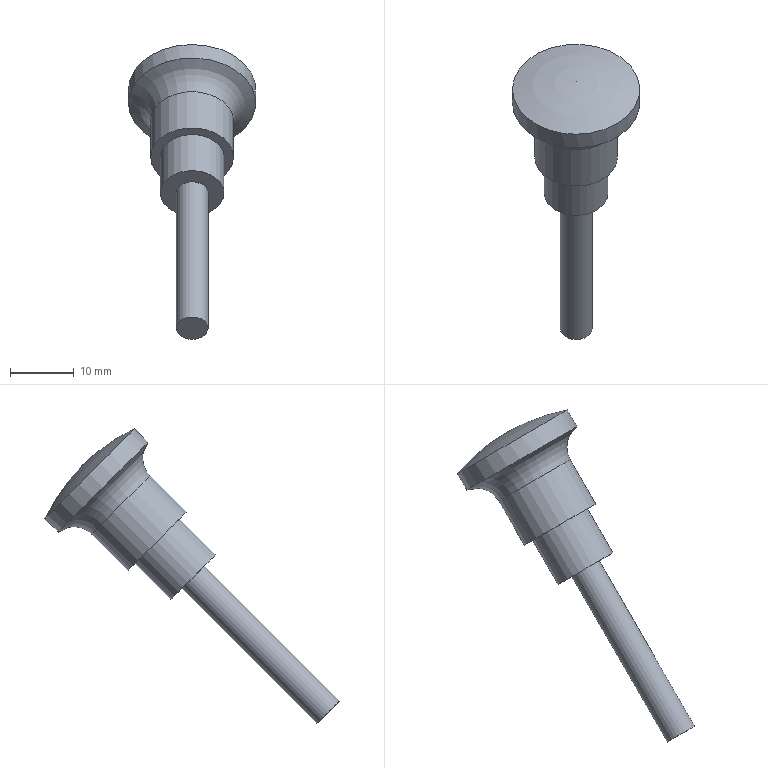Component | NX | YOUBIAO | 1 solid | 9 faces | box 20 x 46.32 x 46.32 mm | volume 4178 mm3 | cylinder 4 | plane 3 | sphere 1 | torus 1 | commonest cylinder face diameters 5 x1 10 x1 20 x1 13 x1
STEP:
#1=CARTESIAN_POINT('',(0.,0.,0.));
#2=DIRECTION('',(0.,0.,1.));
#3=DIRECTION('',(1.,0.,0.));
#4=AXIS2_PLACEMENT_3D('',#1,#2,#3);
#5=CARTESIAN_POINT('',(2.5,317.929,-155.071));
#6=VERTEX_POINT('',#5);
#7=CARTESIAN_POINT('',(0.,317.929,-155.071));
#8=DIRECTION('',(0.,0.7071,0.7071));
#9=DIRECTION('',(1.,0.,0.));
#10=AXIS2_PLACEMENT_3D('',#7,#8,#9);
#11=CIRCLE('',#10,2.5);
#12=CARTESIAN_POINT('',(0.,317.929,-155.071));
#13=DIRECTION('',(0.,-0.7071,-0.7071));
#14=DIRECTION('',(-1.,0.,0.));
#15=AXIS2_PLACEMENT_3D('',#12,#13,#14);
#16=CYLINDRICAL_SURFACE('',#15,2.5);
#17=CARTESIAN_POINT('',(9.425,0.));
#18=DIRECTION('',(-1.,0.));
#19=VECTOR('',#18,1.);
#20=LINE('',#17,#19);
#21=(GEOMETRIC_REPRESENTATION_CONTEXT(2)PARAMETRIC_REPRESENTATION_CONTEXT()REPRESENTATION_CONTEXT('',''));
#22=DEFINITIONAL_REPRESENTATION('',(#20),#21);
#23=PCURVE('',#16,#22);
#24=CARTESIAN_POINT('',(0.,317.929,-155.071));
#25=DIRECTION('',(0.,0.7071,0.7071));
#26=DIRECTION('',(1.,0.,0.));
#27=AXIS2_PLACEMENT_3D('',#24,#25,#26);
#28=PLANE('',#27);
#29=CARTESIAN_POINT('',(0.,0.));
#30=DIRECTION('',(1.,0.));
#31=AXIS2_PLACEMENT_2D('',#29,#30);
#32=CIRCLE('',#31,2.5);
#33=(GEOMETRIC_REPRESENTATION_CONTEXT(2)PARAMETRIC_REPRESENTATION_CONTEXT()REPRESENTATION_CONTEXT('',''));
#34=DEFINITIONAL_REPRESENTATION('',(#32),#33);
#35=PCURVE('',#28,#34);
#36=SURFACE_CURVE('',#11,(#23,#35),.PCURVE_S1.);
#37=EDGE_CURVE('',#6,#6,#36,.T.);
#38=ORIENTED_EDGE('',*,*,#37,.F.);
#39=CARTESIAN_POINT('',(2.5,296.716,-176.284));
#40=VERTEX_POINT('',#39);
#41=CARTESIAN_POINT('',(2.5,317.929,-155.071));
#42=CARTESIAN_POINT('',(2.5,296.716,-176.284));
#43=B_SPLINE_CURVE_WITH_KNOTS('',1,(#41,#42),.UNSPECIFIED.,.F.,.F.,(2,2),(0.,30.),.PIECEWISE_BEZIER_KNOTS.);
#44=CARTESIAN_POINT('',(9.425,0.));
#45=DIRECTION('',(0.,1.));
#46=VECTOR('',#45,1.);
#47=LINE('',#44,#46);
#48=(GEOMETRIC_REPRESENTATION_CONTEXT(2)PARAMETRIC_REPRESENTATION_CONTEXT()REPRESENTATION_CONTEXT('',''));
#49=DEFINITIONAL_REPRESENTATION('',(#47),#48);
#50=PCURVE('',#16,#49);
#51=CARTESIAN_POINT('',(3.142,0.));
#52=DIRECTION('',(0.,1.));
#53=VECTOR('',#52,1.);
#54=LINE('',#51,#53);
#55=(GEOMETRIC_REPRESENTATION_CONTEXT(2)PARAMETRIC_REPRESENTATION_CONTEXT()REPRESENTATION_CONTEXT('',''));
#56=DEFINITIONAL_REPRESENTATION('',(#54),#55);
#57=PCURVE('',#16,#56);
#58=SEAM_CURVE('',#43,(#50,#57),.PCURVE_S1.);
#59=EDGE_CURVE('',#6,#40,#58,.T.);
#60=ORIENTED_EDGE('',*,*,#59,.T.);
#61=CARTESIAN_POINT('',(0.,296.716,-176.284));
#62=DIRECTION('',(0.,0.7071,0.7071));
#63=DIRECTION('',(1.,0.,0.));
#64=AXIS2_PLACEMENT_3D('',#61,#62,#63);
#65=CIRCLE('',#64,2.5);
#66=CARTESIAN_POINT('',(9.425,30.));
#67=DIRECTION('',(-1.,0.));
#68=VECTOR('',#67,1.);
#69=LINE('',#66,#68);
#70=(GEOMETRIC_REPRESENTATION_CONTEXT(2)PARAMETRIC_REPRESENTATION_CONTEXT()REPRESENTATION_CONTEXT('',''));
#71=DEFINITIONAL_REPRESENTATION('',(#69),#70);
#72=PCURVE('',#16,#71);
#73=CARTESIAN_POINT('',(0.,296.716,-176.284));
#74=DIRECTION('',(0.,0.7071,0.7071));
#75=DIRECTION('',(1.,0.,0.));
#76=AXIS2_PLACEMENT_3D('',#73,#74,#75);
#77=PLANE('',#76);
#78=CARTESIAN_POINT('',(0.,0.));
#79=DIRECTION('',(1.,0.));
#80=AXIS2_PLACEMENT_2D('',#78,#79);
#81=CIRCLE('',#80,2.5);
#82=(GEOMETRIC_REPRESENTATION_CONTEXT(2)PARAMETRIC_REPRESENTATION_CONTEXT()REPRESENTATION_CONTEXT('',''));
#83=DEFINITIONAL_REPRESENTATION('',(#81),#82);
#84=PCURVE('',#77,#83);
#85=SURFACE_CURVE('',#65,(#72,#84),.PCURVE_S1.);
#86=EDGE_CURVE('',#40,#40,#85,.T.);
#87=ORIENTED_EDGE('',*,*,#86,.T.);
#88=ORIENTED_EDGE('',*,*,#59,.F.);
#89=EDGE_LOOP('',(#38,#60,#87,#88));
#90=FACE_BOUND('',#89,.T.);
#91=ADVANCED_FACE('',(#90),#16,.T.);
#92=ORIENTED_EDGE('',*,*,#86,.F.);
#93=EDGE_LOOP('',(#92));
#94=FACE_BOUND('',#93,.T.);
#95=ADVANCED_FACE('',(#94),#77,.F.);
#96=CARTESIAN_POINT('',(5.,317.929,-155.071));
#97=VERTEX_POINT('',#96);
#98=CARTESIAN_POINT('',(0.,317.929,-155.071));
#99=DIRECTION('',(0.,0.7071,0.7071));
#100=DIRECTION('',(1.,0.,0.));
#101=AXIS2_PLACEMENT_3D('',#98,#99,#100);
#102=CIRCLE('',#101,5.);
#103=CARTESIAN_POINT('',(0.,0.));
#104=DIRECTION('',(1.,0.));
#105=AXIS2_PLACEMENT_2D('',#103,#104);
#106=CIRCLE('',#105,5.);
#107=(GEOMETRIC_REPRESENTATION_CONTEXT(2)PARAMETRIC_REPRESENTATION_CONTEXT()REPRESENTATION_CONTEXT('',''));
#108=DEFINITIONAL_REPRESENTATION('',(#106),#107);
#109=PCURVE('',#28,#108);
#110=CARTESIAN_POINT('',(0.,323.586,-149.414));
#111=DIRECTION('',(0.,-0.7071,-0.7071));
#112=DIRECTION('',(-1.,0.,0.));
#113=AXIS2_PLACEMENT_3D('',#110,#111,#112);
#114=CYLINDRICAL_SURFACE('',#113,5.);
#115=CARTESIAN_POINT('',(9.425,8.));
#116=DIRECTION('',(-1.,0.));
#117=VECTOR('',#116,1.);
#118=LINE('',#115,#117);
#119=(GEOMETRIC_REPRESENTATION_CONTEXT(2)PARAMETRIC_REPRESENTATION_CONTEXT()REPRESENTATION_CONTEXT('',''));
#120=DEFINITIONAL_REPRESENTATION('',(#118),#119);
#121=PCURVE('',#114,#120);
#122=SURFACE_CURVE('',#102,(#109,#121),.PCURVE_S1.);
#123=EDGE_CURVE('',#97,#97,#122,.T.);
#124=ORIENTED_EDGE('',*,*,#123,.F.);
#125=EDGE_LOOP('',(#124));
#126=FACE_BOUND('',#125,.T.);
#127=ORIENTED_EDGE('',*,*,#37,.T.);
#128=EDGE_LOOP('',(#127));
#129=FACE_BOUND('',#128,.T.);
#130=ADVANCED_FACE('',(#126,#129),#28,.F.);
#131=CARTESIAN_POINT('',(5.,323.586,-149.414));
#132=VERTEX_POINT('',#131);
#133=CARTESIAN_POINT('',(0.,323.586,-149.414));
#134=DIRECTION('',(0.,0.7071,0.7071));
#135=DIRECTION('',(1.,0.,0.));
#136=AXIS2_PLACEMENT_3D('',#133,#134,#135);
#137=CIRCLE('',#136,5.);
#138=CARTESIAN_POINT('',(9.425,0.));
#139=DIRECTION('',(-1.,0.));
#140=VECTOR('',#139,1.);
#141=LINE('',#138,#140);
#142=(GEOMETRIC_REPRESENTATION_CONTEXT(2)PARAMETRIC_REPRESENTATION_CONTEXT()REPRESENTATION_CONTEXT('',''));
#143=DEFINITIONAL_REPRESENTATION('',(#141),#142);
#144=PCURVE('',#114,#143);
#145=CARTESIAN_POINT('',(0.,323.586,-149.414));
#146=DIRECTION('',(0.,-0.7071,-0.7071));
#147=DIRECTION('',(-1.,0.,0.));
#148=AXIS2_PLACEMENT_3D('',#145,#146,#147);
#149=PLANE('',#148);
#150=CARTESIAN_POINT('',(-5.,0.));
#151=CARTESIAN_POINT('',(-5.,8.66));
#152=CARTESIAN_POINT('',(2.5,4.33));
#153=CARTESIAN_POINT('',(10.,0.));
#154=CARTESIAN_POINT('',(2.5,-4.33));
#155=CARTESIAN_POINT('',(-5.,-8.66));
#156=CARTESIAN_POINT('',(-5.,0.));
#157=(BOUNDED_CURVE()B_SPLINE_CURVE(2,(#150,#151,#152,#153,#154,#155,#156),.UNSPECIFIED.,.T.,.F.)B_SPLINE_CURVE_WITH_KNOTS((1,2,2,2,2,1),(-2.094,0.,2.094,4.189,6.283,8.378),.UNSPECIFIED.)CURVE()GEOMETRIC_REPRESENTATION_ITEM()RATIONAL_B_SPLINE_CURVE((1.,0.5,1.,0.5,1.,0.5,1.))REPRESENTATION_ITEM(''));
#158=(GEOMETRIC_REPRESENTATION_CONTEXT(2)PARAMETRIC_REPRESENTATION_CONTEXT()REPRESENTATION_CONTEXT('',''));
#159=DEFINITIONAL_REPRESENTATION('',(#157),#158);
#160=PCURVE('',#149,#159);
#161=SURFACE_CURVE('',#137,(#144,#160),.PCURVE_S1.);
#162=EDGE_CURVE('',#132,#132,#161,.T.);
#163=ORIENTED_EDGE('',*,*,#162,.F.);
#164=CARTESIAN_POINT('',(5.,323.586,-149.414));
#165=CARTESIAN_POINT('',(5.,317.929,-155.071));
#166=B_SPLINE_CURVE_WITH_KNOTS('',1,(#164,#165),.UNSPECIFIED.,.F.,.F.,(2,2),(0.,8.),.PIECEWISE_BEZIER_KNOTS.);
#167=CARTESIAN_POINT('',(9.425,0.));
#168=DIRECTION('',(0.,1.));
#169=VECTOR('',#168,1.);
#170=LINE('',#167,#169);
#171=(GEOMETRIC_REPRESENTATION_CONTEXT(2)PARAMETRIC_REPRESENTATION_CONTEXT()REPRESENTATION_CONTEXT('',''));
#172=DEFINITIONAL_REPRESENTATION('',(#170),#171);
#173=PCURVE('',#114,#172);
#174=CARTESIAN_POINT('',(3.142,0.));
#175=DIRECTION('',(0.,1.));
#176=VECTOR('',#175,1.);
#177=LINE('',#174,#176);
#178=(GEOMETRIC_REPRESENTATION_CONTEXT(2)PARAMETRIC_REPRESENTATION_CONTEXT()REPRESENTATION_CONTEXT('',''));
#179=DEFINITIONAL_REPRESENTATION('',(#177),#178);
#180=PCURVE('',#114,#179);
#181=SEAM_CURVE('',#166,(#173,#180),.PCURVE_S1.);
#182=EDGE_CURVE('',#132,#97,#181,.T.);
#183=ORIENTED_EDGE('',*,*,#182,.T.);
#184=ORIENTED_EDGE('',*,*,#123,.T.);
#185=ORIENTED_EDGE('',*,*,#182,.F.);
#186=EDGE_LOOP('',(#163,#183,#184,#185));
#187=FACE_BOUND('',#186,.T.);
#188=ADVANCED_FACE('',(#187),#114,.T.);
#189=ORIENTED_EDGE('',*,*,#162,.T.);
#190=EDGE_LOOP('',(#189));
#191=FACE_BOUND('',#190,.T.);
#192=CARTESIAN_POINT('',(-6.5,323.586,-149.414));
#193=VERTEX_POINT('',#192);
#194=CARTESIAN_POINT('',(0.,323.586,-149.414));
#195=DIRECTION('',(0.,-0.7071,-0.7071));
#196=DIRECTION('',(-1.,0.,0.));
#197=AXIS2_PLACEMENT_3D('',#194,#195,#196);
#198=CIRCLE('',#197,6.5);
#199=CARTESIAN_POINT('',(0.,0.));
#200=DIRECTION('',(1.,0.));
#201=AXIS2_PLACEMENT_2D('',#199,#200);
#202=CIRCLE('',#201,6.5);
#203=(GEOMETRIC_REPRESENTATION_CONTEXT(2)PARAMETRIC_REPRESENTATION_CONTEXT()REPRESENTATION_CONTEXT('',''));
#204=DEFINITIONAL_REPRESENTATION('',(#202),#203);
#205=PCURVE('',#149,#204);
#206=CARTESIAN_POINT('',(0.,323.586,-149.414));
#207=DIRECTION('',(0.,-0.7071,-0.7071));
#208=DIRECTION('',(-1.,0.,0.));
#209=AXIS2_PLACEMENT_3D('',#206,#207,#208);
#210=CYLINDRICAL_SURFACE('',#209,6.5);
#211=CARTESIAN_POINT('',(0.,0.));
#212=DIRECTION('',(1.,0.));
#213=VECTOR('',#212,1.);
#214=LINE('',#211,#213);
#215=(GEOMETRIC_REPRESENTATION_CONTEXT(2)PARAMETRIC_REPRESENTATION_CONTEXT()REPRESENTATION_CONTEXT('',''));
#216=DEFINITIONAL_REPRESENTATION('',(#214),#215);
#217=PCURVE('',#210,#216);
#218=SURFACE_CURVE('',#198,(#205,#217),.PCURVE_S1.);
#219=EDGE_CURVE('',#193,#193,#218,.T.);
#220=ORIENTED_EDGE('',*,*,#219,.T.);
#221=EDGE_LOOP('',(#220));
#222=FACE_BOUND('',#221,.T.);
#223=ADVANCED_FACE('',(#191,#222),#149,.T.);
#224=CARTESIAN_POINT('',(0.,327.121,-131.737));
#225=VERTEX_POINT('',#224);
#226=CARTESIAN_POINT('',(-10.,334.192,-138.808));
#227=VERTEX_POINT('',#226);
#228=CARTESIAN_POINT('',(0.,334.192,-138.808));
#229=DIRECTION('',(0.,-0.7071,-0.7071));
#230=DIRECTION('',(-1.,0.,0.));
#231=AXIS2_PLACEMENT_3D('',#228,#229,#230);
#232=CIRCLE('',#231,10.);
#233=CARTESIAN_POINT('',(0.,314.192,-158.808));
#234=DIRECTION('',(0.,-0.7071,-0.7071));
#235=DIRECTION('',(0.,-0.7071,0.7071));
#236=AXIS2_PLACEMENT_3D('',#233,#234,#235);
#237=SPHERICAL_SURFACE('',#236,30.);
#238=CARTESIAN_POINT('',(-4.712,-1.231));
#239=CARTESIAN_POINT('',(-4.617,-1.231));
#240=CARTESIAN_POINT('',(-4.427,-1.231));
#241=CARTESIAN_POINT('',(-4.141,-1.231));
#242=CARTESIAN_POINT('',(-3.856,-1.231));
#243=CARTESIAN_POINT('',(-3.57,-1.231));
#244=CARTESIAN_POINT('',(-3.284,-1.231));
#245=CARTESIAN_POINT('',(-2.999,-1.231));
#246=CARTESIAN_POINT('',(-2.713,-1.231));
#247=CARTESIAN_POINT('',(-2.428,-1.231));
#248=CARTESIAN_POINT('',(-2.142,-1.231));
#249=CARTESIAN_POINT('',(-1.856,-1.231));
#250=CARTESIAN_POINT('',(-1.571,-1.231));
#251=CARTESIAN_POINT('',(-1.285,-1.231));
#252=CARTESIAN_POINT('',(-0.9996,-1.231));
#253=CARTESIAN_POINT('',(-0.714,-1.231));
#254=CARTESIAN_POINT('',(-0.4284,-1.231));
#255=CARTESIAN_POINT('',(-0.1428,-1.231));
#256=CARTESIAN_POINT('',(0.1428,-1.231));
#257=CARTESIAN_POINT('',(0.4284,-1.231));
#258=CARTESIAN_POINT('',(0.714,-1.231));
#259=CARTESIAN_POINT('',(0.9996,-1.231));
#260=CARTESIAN_POINT('',(1.285,-1.231));
#261=CARTESIAN_POINT('',(1.476,-1.231));
#262=CARTESIAN_POINT('',(1.571,-1.231));
#263=B_SPLINE_CURVE_WITH_KNOTS('',3,(#238,#239,#240,#241,#242,#243,#244,#245,#246,#247,#248,#249,#250,#251,#252,#253,#254,#255,#256,#257,#258,#259,#260,#261,#262),.UNSPECIFIED.,.F.,.F.,(4,1,1,1,1,1,1,1,1,1,1,1,1,1,1,1,1,1,1,1,1,1,4),(0.,0.2856,0.5712,0.8568,1.142,1.428,1.714,1.999,2.285,2.57,2.856,3.142,3.427,3.713,3.998,4.284,4.57,4.855,5.141,5.426,5.712,5.998,6.283),.QUASI_UNIFORM_KNOTS.);
#264=(GEOMETRIC_REPRESENTATION_CONTEXT(2)PARAMETRIC_REPRESENTATION_CONTEXT()REPRESENTATION_CONTEXT('',''));
#265=DEFINITIONAL_REPRESENTATION('',(#263),#264);
#266=PCURVE('',#237,#265);
#267=CARTESIAN_POINT('',(0.,323.586,-149.414));
#268=DIRECTION('',(0.,-0.7071,-0.7071));
#269=DIRECTION('',(-1.,0.,0.));
#270=AXIS2_PLACEMENT_3D('',#267,#268,#269);
#271=CYLINDRICAL_SURFACE('',#270,10.);
#272=CARTESIAN_POINT('',(0.,-15.));
#273=DIRECTION('',(1.,0.));
#274=VECTOR('',#273,1.);
#275=LINE('',#272,#274);
#276=(GEOMETRIC_REPRESENTATION_CONTEXT(2)PARAMETRIC_REPRESENTATION_CONTEXT()REPRESENTATION_CONTEXT('',''));
#277=DEFINITIONAL_REPRESENTATION('',(#275),#276);
#278=PCURVE('',#271,#277);
#279=SURFACE_CURVE('',#232,(#266,#278),.PCURVE_S1.);
#280=EDGE_CURVE('',#225,#227,#279,.T.);
#281=ORIENTED_EDGE('',*,*,#280,.F.);
#282=CARTESIAN_POINT('',(0.,335.406,-137.594));
#283=VERTEX_POINT('',#282);
#284=CARTESIAN_POINT('',(0.,335.406,-137.594));
#285=CARTESIAN_POINT('',(0.,333.964,-136.153));
#286=CARTESIAN_POINT('',(0.,332.399,-134.833));
#287=CARTESIAN_POINT('',(0.,330.727,-133.65));
#288=CARTESIAN_POINT('',(0.,328.961,-132.615));
#289=CARTESIAN_POINT('',(0.,327.121,-131.737));
#290=B_SPLINE_CURVE_WITH_KNOTS('',5,(#284,#285,#286,#287,#288,#289),.UNSPECIFIED.,.F.,.F.,(6,6),(-1.571,-1.231),.PIECEWISE_BEZIER_KNOTS.);
#291=CARTESIAN_POINT('',(0.,0.));
#292=DIRECTION('',(0.,1.));
#293=VECTOR('',#292,1.);
#294=LINE('',#291,#293);
#295=(GEOMETRIC_REPRESENTATION_CONTEXT(2)PARAMETRIC_REPRESENTATION_CONTEXT()REPRESENTATION_CONTEXT('',''));
#296=DEFINITIONAL_REPRESENTATION('',(#294),#295);
#297=PCURVE('',#237,#296);
#298=CARTESIAN_POINT('',(6.283,0.));
#299=DIRECTION('',(0.,1.));
#300=VECTOR('',#299,1.);
#301=LINE('',#298,#300);
#302=(GEOMETRIC_REPRESENTATION_CONTEXT(2)PARAMETRIC_REPRESENTATION_CONTEXT()REPRESENTATION_CONTEXT('',''));
#303=DEFINITIONAL_REPRESENTATION('',(#301),#302);
#304=PCURVE('',#237,#303);
#305=SEAM_CURVE('',#290,(#297,#304),.PCURVE_S1.);
#306=EDGE_CURVE('',#283,#225,#305,.T.);
#307=ORIENTED_EDGE('',*,*,#306,.F.);
#308=ORIENTED_EDGE('',*,*,#306,.T.);
#309=CARTESIAN_POINT('',(0.,334.192,-138.808));
#310=DIRECTION('',(0.,-0.7071,-0.7071));
#311=DIRECTION('',(-1.,0.,0.));
#312=AXIS2_PLACEMENT_3D('',#309,#310,#311);
#313=CIRCLE('',#312,10.);
#314=CARTESIAN_POINT('',(1.571,-1.231));
#315=CARTESIAN_POINT('',(1.666,-1.231));
#316=CARTESIAN_POINT('',(1.856,-1.231));
#317=CARTESIAN_POINT('',(2.142,-1.231));
#318=CARTESIAN_POINT('',(2.428,-1.231));
#319=CARTESIAN_POINT('',(2.713,-1.231));
#320=CARTESIAN_POINT('',(2.999,-1.231));
#321=CARTESIAN_POINT('',(3.284,-1.231));
#322=CARTESIAN_POINT('',(3.57,-1.231));
#323=CARTESIAN_POINT('',(3.856,-1.231));
#324=CARTESIAN_POINT('',(4.141,-1.231));
#325=CARTESIAN_POINT('',(4.427,-1.231));
#326=CARTESIAN_POINT('',(4.712,-1.231));
#327=CARTESIAN_POINT('',(4.998,-1.231));
#328=CARTESIAN_POINT('',(5.284,-1.231));
#329=CARTESIAN_POINT('',(5.569,-1.231));
#330=CARTESIAN_POINT('',(5.855,-1.231));
#331=CARTESIAN_POINT('',(6.14,-1.231));
#332=CARTESIAN_POINT('',(6.426,-1.231));
#333=CARTESIAN_POINT('',(6.712,-1.231));
#334=CARTESIAN_POINT('',(6.997,-1.231));
#335=CARTESIAN_POINT('',(7.283,-1.231));
#336=CARTESIAN_POINT('',(7.568,-1.231));
#337=CARTESIAN_POINT('',(7.759,-1.231));
#338=CARTESIAN_POINT('',(7.854,-1.231));
#339=B_SPLINE_CURVE_WITH_KNOTS('',3,(#314,#315,#316,#317,#318,#319,#320,#321,#322,#323,#324,#325,#326,#327,#328,#329,#330,#331,#332,#333,#334,#335,#336,#337,#338),.UNSPECIFIED.,.F.,.F.,(4,1,1,1,1,1,1,1,1,1,1,1,1,1,1,1,1,1,1,1,1,1,4),(0.,0.2856,0.5712,0.8568,1.142,1.428,1.714,1.999,2.285,2.57,2.856,3.142,3.427,3.713,3.998,4.284,4.57,4.855,5.141,5.426,5.712,5.998,6.283),.QUASI_UNIFORM_KNOTS.);
#340=(GEOMETRIC_REPRESENTATION_CONTEXT(2)PARAMETRIC_REPRESENTATION_CONTEXT()REPRESENTATION_CONTEXT('',''));
#341=DEFINITIONAL_REPRESENTATION('',(#339),#340);
#342=PCURVE('',#237,#341);
#343=CARTESIAN_POINT('',(0.,-15.));
#344=DIRECTION('',(1.,0.));
#345=VECTOR('',#344,1.);
#346=LINE('',#343,#345);
#347=(GEOMETRIC_REPRESENTATION_CONTEXT(2)PARAMETRIC_REPRESENTATION_CONTEXT()REPRESENTATION_CONTEXT('',''));
#348=DEFINITIONAL_REPRESENTATION('',(#346),#347);
#349=PCURVE('',#271,#348);
#350=SURFACE_CURVE('',#313,(#342,#349),.PCURVE_S1.);
#351=EDGE_CURVE('',#227,#225,#350,.T.);
#352=ORIENTED_EDGE('',*,*,#351,.F.);
#353=EDGE_LOOP('',(#281,#307,#308,#352));
#354=FACE_BOUND('',#353,.T.);
#355=ADVANCED_FACE('',(#354),#237,.T.);
#356=ORIENTED_EDGE('',*,*,#351,.T.);
#357=ORIENTED_EDGE('',*,*,#280,.T.);
#358=CARTESIAN_POINT('',(-10.,332.071,-140.929));
#359=VERTEX_POINT('',#358);
#360=CARTESIAN_POINT('',(-10.,334.192,-138.808));
#361=CARTESIAN_POINT('',(-10.,332.071,-140.929));
#362=B_SPLINE_CURVE_WITH_KNOTS('',1,(#360,#361),.UNSPECIFIED.,.F.,.F.,(2,2),(-15.,-12.),.PIECEWISE_BEZIER_KNOTS.);
#363=CARTESIAN_POINT('',(6.283,0.));
#364=DIRECTION('',(0.,1.));
#365=VECTOR('',#364,1.);
#366=LINE('',#363,#365);
#367=(GEOMETRIC_REPRESENTATION_CONTEXT(2)PARAMETRIC_REPRESENTATION_CONTEXT()REPRESENTATION_CONTEXT('',''));
#368=DEFINITIONAL_REPRESENTATION('',(#366),#367);
#369=PCURVE('',#271,#368);
#370=CARTESIAN_POINT('',(0.,0.));
#371=DIRECTION('',(0.,1.));
#372=VECTOR('',#371,1.);
#373=LINE('',#370,#372);
#374=(GEOMETRIC_REPRESENTATION_CONTEXT(2)PARAMETRIC_REPRESENTATION_CONTEXT()REPRESENTATION_CONTEXT('',''));
#375=DEFINITIONAL_REPRESENTATION('',(#373),#374);
#376=PCURVE('',#271,#375);
#377=SEAM_CURVE('',#362,(#369,#376),.PCURVE_S1.);
#378=EDGE_CURVE('',#227,#359,#377,.T.);
#379=ORIENTED_EDGE('',*,*,#378,.T.);
#380=CARTESIAN_POINT('',(0.,332.071,-140.929));
#381=DIRECTION('',(0.,-0.7071,-0.7071));
#382=DIRECTION('',(-1.,0.,0.));
#383=AXIS2_PLACEMENT_3D('',#380,#381,#382);
#384=CIRCLE('',#383,10.);
#385=CARTESIAN_POINT('',(0.,-12.));
#386=DIRECTION('',(1.,0.));
#387=VECTOR('',#386,1.);
#388=LINE('',#385,#387);
#389=(GEOMETRIC_REPRESENTATION_CONTEXT(2)PARAMETRIC_REPRESENTATION_CONTEXT()REPRESENTATION_CONTEXT('',''));
#390=DEFINITIONAL_REPRESENTATION('',(#388),#389);
#391=PCURVE('',#271,#390);
#392=CARTESIAN_POINT('',(0.,329.265,-143.735));
#393=DIRECTION('',(0.,-0.7071,-0.7071));
#394=DIRECTION('',(-1.,0.,0.));
#395=AXIS2_PLACEMENT_3D('',#392,#393,#394);
#396=TOROIDAL_SURFACE('',#395,10.5,4.);
#397=CARTESIAN_POINT('',(0.,4.587));
#398=DIRECTION('',(1.,0.));
#399=VECTOR('',#398,1.);
#400=LINE('',#397,#399);
#401=(GEOMETRIC_REPRESENTATION_CONTEXT(2)PARAMETRIC_REPRESENTATION_CONTEXT()REPRESENTATION_CONTEXT('',''));
#402=DEFINITIONAL_REPRESENTATION('',(#400),#401);
#403=PCURVE('',#396,#402);
#404=SURFACE_CURVE('',#384,(#391,#403),.PCURVE_S1.);
#405=EDGE_CURVE('',#359,#359,#404,.T.);
#406=ORIENTED_EDGE('',*,*,#405,.F.);
#407=ORIENTED_EDGE('',*,*,#378,.F.);
#408=EDGE_LOOP('',(#356,#357,#379,#406,#407));
#409=FACE_BOUND('',#408,.T.);
#410=ADVANCED_FACE('',(#409),#271,.T.);
#411=ORIENTED_EDGE('',*,*,#405,.F.);
#412=CARTESIAN_POINT('',(-6.5,329.265,-143.735));
#413=VERTEX_POINT('',#412);
#414=CARTESIAN_POINT('',(-6.5,329.265,-143.735));
#415=CARTESIAN_POINT('',(-6.5,329.958,-143.042));
#416=CARTESIAN_POINT('',(-6.786,330.637,-142.363));
#417=CARTESIAN_POINT('',(-7.34,331.236,-141.764));
#418=CARTESIAN_POINT('',(-8.111,331.699,-141.301));
#419=CARTESIAN_POINT('',(-9.027,331.984,-141.016));
#420=CARTESIAN_POINT('',(-10.,332.071,-140.929));
#421=(BOUNDED_CURVE()B_SPLINE_CURVE(6,(#414,#415,#416,#417,#418,#419,#420),.UNSPECIFIED.,.F.,.F.)B_SPLINE_CURVE_WITH_KNOTS((7,7),(3.142,4.587),.PIECEWISE_BEZIER_KNOTS.)CURVE()GEOMETRIC_REPRESENTATION_ITEM()RATIONAL_B_SPLINE_CURVE((1.027,1.009,0.9982,0.9949,0.9982,1.009,1.027))REPRESENTATION_ITEM(''));
#422=CARTESIAN_POINT('',(0.,0.));
#423=DIRECTION('',(0.,1.));
#424=VECTOR('',#423,1.);
#425=LINE('',#422,#424);
#426=(GEOMETRIC_REPRESENTATION_CONTEXT(2)PARAMETRIC_REPRESENTATION_CONTEXT()REPRESENTATION_CONTEXT('',''));
#427=DEFINITIONAL_REPRESENTATION('',(#425),#426);
#428=PCURVE('',#396,#427);
#429=CARTESIAN_POINT('',(6.283,0.));
#430=DIRECTION('',(0.,1.));
#431=VECTOR('',#430,1.);
#432=LINE('',#429,#431);
#433=(GEOMETRIC_REPRESENTATION_CONTEXT(2)PARAMETRIC_REPRESENTATION_CONTEXT()REPRESENTATION_CONTEXT('',''));
#434=DEFINITIONAL_REPRESENTATION('',(#432),#433);
#435=PCURVE('',#396,#434);
#436=SEAM_CURVE('',#421,(#428,#435),.PCURVE_S1.);
#437=EDGE_CURVE('',#413,#359,#436,.T.);
#438=ORIENTED_EDGE('',*,*,#437,.F.);
#439=CARTESIAN_POINT('',(0.,329.265,-143.735));
#440=DIRECTION('',(0.,-0.7071,-0.7071));
#441=DIRECTION('',(-1.,0.,0.));
#442=AXIS2_PLACEMENT_3D('',#439,#440,#441);
#443=CIRCLE('',#442,6.5);
#444=CARTESIAN_POINT('',(0.,3.142));
#445=DIRECTION('',(1.,0.));
#446=VECTOR('',#445,1.);
#447=LINE('',#444,#446);
#448=(GEOMETRIC_REPRESENTATION_CONTEXT(2)PARAMETRIC_REPRESENTATION_CONTEXT()REPRESENTATION_CONTEXT('',''));
#449=DEFINITIONAL_REPRESENTATION('',(#447),#448);
#450=PCURVE('',#396,#449);
#451=CARTESIAN_POINT('',(0.,-8.031));
#452=DIRECTION('',(1.,0.));
#453=VECTOR('',#452,1.);
#454=LINE('',#451,#453);
#455=(GEOMETRIC_REPRESENTATION_CONTEXT(2)PARAMETRIC_REPRESENTATION_CONTEXT()REPRESENTATION_CONTEXT('',''));
#456=DEFINITIONAL_REPRESENTATION('',(#454),#455);
#457=PCURVE('',#210,#456);
#458=SURFACE_CURVE('',#443,(#450,#457),.PCURVE_S1.);
#459=EDGE_CURVE('',#413,#413,#458,.T.);
#460=ORIENTED_EDGE('',*,*,#459,.T.);
#461=ORIENTED_EDGE('',*,*,#437,.T.);
#462=EDGE_LOOP('',(#411,#438,#460,#461));
#463=FACE_BOUND('',#462,.F.);
#464=ADVANCED_FACE('',(#463),#396,.F.);
#465=ORIENTED_EDGE('',*,*,#459,.T.);
#466=CARTESIAN_POINT('',(-6.5,329.265,-143.735));
#467=CARTESIAN_POINT('',(-6.5,323.586,-149.414));
#468=B_SPLINE_CURVE_WITH_KNOTS('',1,(#466,#467),.UNSPECIFIED.,.F.,.F.,(2,2),(-8.031,0.),.PIECEWISE_BEZIER_KNOTS.);
#469=CARTESIAN_POINT('',(6.283,0.));
#470=DIRECTION('',(0.,1.));
#471=VECTOR('',#470,1.);
#472=LINE('',#469,#471);
#473=(GEOMETRIC_REPRESENTATION_CONTEXT(2)PARAMETRIC_REPRESENTATION_CONTEXT()REPRESENTATION_CONTEXT('',''));
#474=DEFINITIONAL_REPRESENTATION('',(#472),#473);
#475=PCURVE('',#210,#474);
#476=CARTESIAN_POINT('',(0.,0.));
#477=DIRECTION('',(0.,1.));
#478=VECTOR('',#477,1.);
#479=LINE('',#476,#478);
#480=(GEOMETRIC_REPRESENTATION_CONTEXT(2)PARAMETRIC_REPRESENTATION_CONTEXT()REPRESENTATION_CONTEXT('',''));
#481=DEFINITIONAL_REPRESENTATION('',(#479),#480);
#482=PCURVE('',#210,#481);
#483=SEAM_CURVE('',#468,(#475,#482),.PCURVE_S1.);
#484=EDGE_CURVE('',#413,#193,#483,.T.);
#485=ORIENTED_EDGE('',*,*,#484,.T.);
#486=ORIENTED_EDGE('',*,*,#219,.F.);
#487=ORIENTED_EDGE('',*,*,#484,.F.);
#488=EDGE_LOOP('',(#465,#485,#486,#487));
#489=FACE_BOUND('',#488,.T.);
#490=ADVANCED_FACE('',(#489),#210,.T.);
#491=CLOSED_SHELL('',(#91,#95,#130,#188,#223,#355,#410,#464,#490));
#492=MANIFOLD_SOLID_BREP('',#491);
#493=(LENGTH_UNIT()NAMED_UNIT(*)SI_UNIT(.MILLI.,.METRE.));
#494=UNCERTAINTY_MEASURE_WITH_UNIT(LENGTH_MEASURE(0.00001),#493,'','');
#495=(NAMED_UNIT(*)PLANE_ANGLE_UNIT()SI_UNIT($,.RADIAN.));
#496=(NAMED_UNIT(*)SI_UNIT($,.STERADIAN.)SOLID_ANGLE_UNIT());
#497=(GEOMETRIC_REPRESENTATION_CONTEXT(3)GLOBAL_UNCERTAINTY_ASSIGNED_CONTEXT((#494))GLOBAL_UNIT_ASSIGNED_CONTEXT((#493,#495,#496))REPRESENTATION_CONTEXT('',''));
#498=ADVANCED_BREP_SHAPE_REPRESENTATION('',(#4,#492),#497);